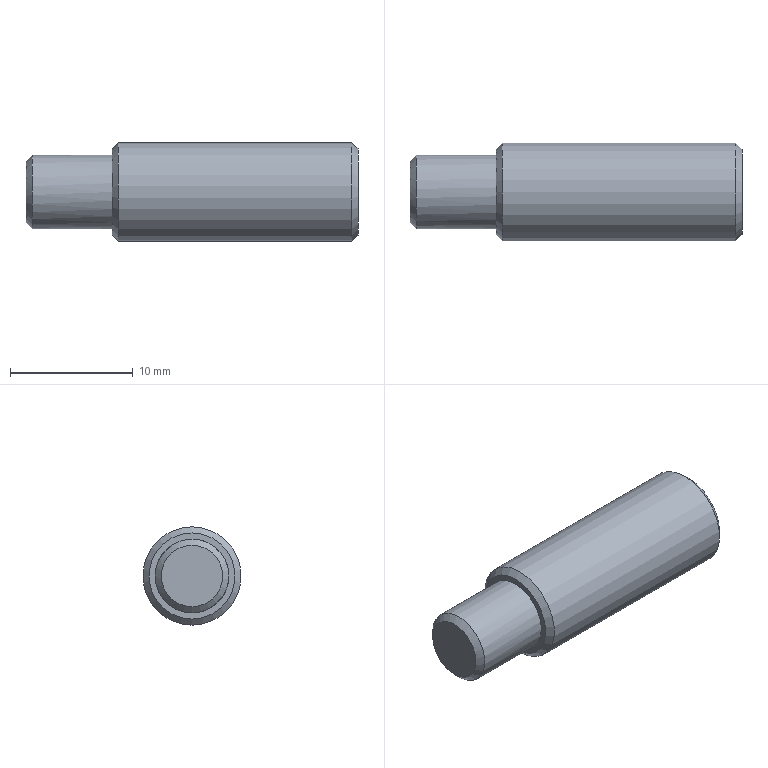Component | NX | LOC_PIN | 1 solid | 8 faces | box 27 x 8 x 8 mm | volume 1195 mm3 | plane 3 | cone 3 | cylinder 2 | commonest cylinder face diameters 6 x1 8 x1
STEP:
#1=CARTESIAN_POINT('',(0.,0.,0.));
#2=DIRECTION('',(0.,0.,1.));
#3=DIRECTION('',(1.,0.,0.));
#4=AXIS2_PLACEMENT_3D('',#1,#2,#3);
#5=CARTESIAN_POINT('',(-29.5,0.,-42.));
#6=VERTEX_POINT('',#5);
#7=CARTESIAN_POINT('',(-29.5,3.,-39.));
#8=VERTEX_POINT('',#7);
#9=CARTESIAN_POINT('',(-29.5,0.,-39.));
#10=DIRECTION('',(1.,0.,0.));
#11=DIRECTION('',(0.,0.,-1.));
#12=AXIS2_PLACEMENT_3D('',#9,#10,#11);
#13=CIRCLE('',#12,3.);
#14=CARTESIAN_POINT('',(-23.,0.,-39.));
#15=DIRECTION('',(-1.,0.,0.));
#16=DIRECTION('',(0.,0.,1.));
#17=AXIS2_PLACEMENT_3D('',#14,#15,#16);
#18=CYLINDRICAL_SURFACE('',#17,3.);
#19=CARTESIAN_POINT('',(3.142,6.5));
#20=DIRECTION('',(-1.,0.));
#21=VECTOR('',#20,1.);
#22=LINE('',#19,#21);
#23=(GEOMETRIC_REPRESENTATION_CONTEXT(2)PARAMETRIC_REPRESENTATION_CONTEXT()REPRESENTATION_CONTEXT('',''));
#24=DEFINITIONAL_REPRESENTATION('',(#22),#23);
#25=PCURVE('',#18,#24);
#26=CARTESIAN_POINT('',(-29.5,0.,-39.));
#27=DIRECTION('',(1.,0.,0.));
#28=DIRECTION('',(0.,0.,-1.));
#29=AXIS2_PLACEMENT_3D('',#26,#27,#28);
#30=CONICAL_SURFACE('',#29,3.,0.7854);
#31=CARTESIAN_POINT('',(0.,0.));
#32=DIRECTION('',(1.,0.));
#33=VECTOR('',#32,1.);
#34=LINE('',#31,#33);
#35=(GEOMETRIC_REPRESENTATION_CONTEXT(2)PARAMETRIC_REPRESENTATION_CONTEXT()REPRESENTATION_CONTEXT('',''));
#36=DEFINITIONAL_REPRESENTATION('',(#34),#35);
#37=PCURVE('',#30,#36);
#38=SURFACE_CURVE('',#13,(#25,#37),.PCURVE_S1.);
#39=EDGE_CURVE('',#6,#8,#38,.T.);
#40=ORIENTED_EDGE('',*,*,#39,.T.);
#41=CARTESIAN_POINT('',(-23.,3.,-39.));
#42=VERTEX_POINT('',#41);
#43=CARTESIAN_POINT('',(-23.,3.,-39.));
#44=CARTESIAN_POINT('',(-29.5,3.,-39.));
#45=B_SPLINE_CURVE_WITH_KNOTS('',1,(#43,#44),.UNSPECIFIED.,.F.,.F.,(2,2),(0.,6.5),.PIECEWISE_BEZIER_KNOTS.);
#46=CARTESIAN_POINT('',(1.571,0.));
#47=DIRECTION('',(0.,1.));
#48=VECTOR('',#47,1.);
#49=LINE('',#46,#48);
#50=(GEOMETRIC_REPRESENTATION_CONTEXT(2)PARAMETRIC_REPRESENTATION_CONTEXT()REPRESENTATION_CONTEXT('',''));
#51=DEFINITIONAL_REPRESENTATION('',(#49),#50);
#52=PCURVE('',#18,#51);
#53=CARTESIAN_POINT('',(7.854,0.));
#54=DIRECTION('',(0.,1.));
#55=VECTOR('',#54,1.);
#56=LINE('',#53,#55);
#57=(GEOMETRIC_REPRESENTATION_CONTEXT(2)PARAMETRIC_REPRESENTATION_CONTEXT()REPRESENTATION_CONTEXT('',''));
#58=DEFINITIONAL_REPRESENTATION('',(#56),#57);
#59=PCURVE('',#18,#58);
#60=SEAM_CURVE('',#45,(#52,#59),.PCURVE_S1.);
#61=EDGE_CURVE('',#42,#8,#60,.T.);
#62=ORIENTED_EDGE('',*,*,#61,.F.);
#63=CARTESIAN_POINT('',(-23.,0.,-39.));
#64=DIRECTION('',(1.,0.,0.));
#65=DIRECTION('',(0.,1.,0.));
#66=AXIS2_PLACEMENT_3D('',#63,#64,#65);
#67=CIRCLE('',#66,3.);
#68=CARTESIAN_POINT('',(7.854,0.));
#69=DIRECTION('',(-1.,0.));
#70=VECTOR('',#69,1.);
#71=LINE('',#68,#70);
#72=(GEOMETRIC_REPRESENTATION_CONTEXT(2)PARAMETRIC_REPRESENTATION_CONTEXT()REPRESENTATION_CONTEXT('',''));
#73=DEFINITIONAL_REPRESENTATION('',(#71),#72);
#74=PCURVE('',#18,#73);
#75=CARTESIAN_POINT('',(-23.,0.,-39.));
#76=DIRECTION('',(1.,0.,0.));
#77=DIRECTION('',(0.,0.,-1.));
#78=AXIS2_PLACEMENT_3D('',#75,#76,#77);
#79=PLANE('',#78);
#80=CARTESIAN_POINT('',(0.,0.));
#81=DIRECTION('',(0.,1.));
#82=AXIS2_PLACEMENT_2D('',#80,#81);
#83=CIRCLE('',#82,3.);
#84=(GEOMETRIC_REPRESENTATION_CONTEXT(2)PARAMETRIC_REPRESENTATION_CONTEXT()REPRESENTATION_CONTEXT('',''));
#85=DEFINITIONAL_REPRESENTATION('',(#83),#84);
#86=PCURVE('',#79,#85);
#87=SURFACE_CURVE('',#67,(#74,#86),.PCURVE_S1.);
#88=EDGE_CURVE('',#42,#42,#87,.T.);
#89=ORIENTED_EDGE('',*,*,#88,.F.);
#90=ORIENTED_EDGE('',*,*,#61,.T.);
#91=CARTESIAN_POINT('',(-29.5,0.,-39.));
#92=DIRECTION('',(1.,0.,0.));
#93=DIRECTION('',(0.,0.,-1.));
#94=AXIS2_PLACEMENT_3D('',#91,#92,#93);
#95=CIRCLE('',#94,3.);
#96=CARTESIAN_POINT('',(9.425,6.5));
#97=DIRECTION('',(-1.,0.));
#98=VECTOR('',#97,1.);
#99=LINE('',#96,#98);
#100=(GEOMETRIC_REPRESENTATION_CONTEXT(2)PARAMETRIC_REPRESENTATION_CONTEXT()REPRESENTATION_CONTEXT('',''));
#101=DEFINITIONAL_REPRESENTATION('',(#99),#100);
#102=PCURVE('',#18,#101);
#103=CARTESIAN_POINT('',(0.,0.));
#104=DIRECTION('',(1.,0.));
#105=VECTOR('',#104,1.);
#106=LINE('',#103,#105);
#107=(GEOMETRIC_REPRESENTATION_CONTEXT(2)PARAMETRIC_REPRESENTATION_CONTEXT()REPRESENTATION_CONTEXT('',''));
#108=DEFINITIONAL_REPRESENTATION('',(#106),#107);
#109=PCURVE('',#30,#108);
#110=SURFACE_CURVE('',#95,(#102,#109),.PCURVE_S1.);
#111=EDGE_CURVE('',#8,#6,#110,.T.);
#112=ORIENTED_EDGE('',*,*,#111,.T.);
#113=EDGE_LOOP('',(#40,#62,#89,#90,#112));
#114=FACE_BOUND('',#113,.T.);
#115=ADVANCED_FACE('',(#114),#18,.T.);
#116=CARTESIAN_POINT('',(-30.,0.,-41.5));
#117=VERTEX_POINT('',#116);
#118=CARTESIAN_POINT('',(-30.,0.,-39.));
#119=DIRECTION('',(-1.,0.,0.));
#120=DIRECTION('',(0.,0.,-1.));
#121=AXIS2_PLACEMENT_3D('',#118,#119,#120);
#122=CIRCLE('',#121,2.5);
#123=CARTESIAN_POINT('',(-30.,0.,-39.));
#124=DIRECTION('',(1.,0.,0.));
#125=DIRECTION('',(0.,0.,-1.));
#126=AXIS2_PLACEMENT_3D('',#123,#124,#125);
#127=PLANE('',#126);
#128=CARTESIAN_POINT('',(2.5,0.));
#129=CARTESIAN_POINT('',(2.5,-4.33));
#130=CARTESIAN_POINT('',(-1.25,-2.165));
#131=CARTESIAN_POINT('',(-5.,-0.));
#132=CARTESIAN_POINT('',(-1.25,2.165));
#133=CARTESIAN_POINT('',(2.5,4.33));
#134=CARTESIAN_POINT('',(2.5,0.));
#135=(BOUNDED_CURVE()B_SPLINE_CURVE(2,(#128,#129,#130,#131,#132,#133,#134),.UNSPECIFIED.,.T.,.F.)B_SPLINE_CURVE_WITH_KNOTS((1,2,2,2,2,1),(-2.094,0.,2.094,4.189,6.283,8.378),.UNSPECIFIED.)CURVE()GEOMETRIC_REPRESENTATION_ITEM()RATIONAL_B_SPLINE_CURVE((1.,0.5,1.,0.5,1.,0.5,1.))REPRESENTATION_ITEM(''));
#136=(GEOMETRIC_REPRESENTATION_CONTEXT(2)PARAMETRIC_REPRESENTATION_CONTEXT()REPRESENTATION_CONTEXT('',''));
#137=DEFINITIONAL_REPRESENTATION('',(#135),#136);
#138=PCURVE('',#127,#137);
#139=CARTESIAN_POINT('',(6.283,-0.5));
#140=DIRECTION('',(-1.,0.));
#141=VECTOR('',#140,1.);
#142=LINE('',#139,#141);
#143=(GEOMETRIC_REPRESENTATION_CONTEXT(2)PARAMETRIC_REPRESENTATION_CONTEXT()REPRESENTATION_CONTEXT('',''));
#144=DEFINITIONAL_REPRESENTATION('',(#142),#143);
#145=PCURVE('',#30,#144);
#146=SURFACE_CURVE('',#122,(#138,#145),.PCURVE_S1.);
#147=EDGE_CURVE('',#117,#117,#146,.T.);
#148=ORIENTED_EDGE('',*,*,#147,.T.);
#149=EDGE_LOOP('',(#148));
#150=FACE_BOUND('',#149,.T.);
#151=ADVANCED_FACE('',(#150),#127,.F.);
#152=CARTESIAN_POINT('',(-22.5,0.,-43.));
#153=VERTEX_POINT('',#152);
#154=CARTESIAN_POINT('',(-22.5,0.,-39.));
#155=DIRECTION('',(1.,0.,0.));
#156=DIRECTION('',(0.,0.,-1.));
#157=AXIS2_PLACEMENT_3D('',#154,#155,#156);
#158=CIRCLE('',#157,4.);
#159=CARTESIAN_POINT('',(-3.,0.,-39.));
#160=DIRECTION('',(-1.,0.,0.));
#161=DIRECTION('',(0.,0.,1.));
#162=AXIS2_PLACEMENT_3D('',#159,#160,#161);
#163=CYLINDRICAL_SURFACE('',#162,4.);
#164=CARTESIAN_POINT('',(9.425,19.5));
#165=DIRECTION('',(-1.,0.));
#166=VECTOR('',#165,1.);
#167=LINE('',#164,#166);
#168=(GEOMETRIC_REPRESENTATION_CONTEXT(2)PARAMETRIC_REPRESENTATION_CONTEXT()REPRESENTATION_CONTEXT('',''));
#169=DEFINITIONAL_REPRESENTATION('',(#167),#168);
#170=PCURVE('',#163,#169);
#171=CARTESIAN_POINT('',(-22.5,0.,-39.));
#172=DIRECTION('',(1.,0.,0.));
#173=DIRECTION('',(0.,0.,-1.));
#174=AXIS2_PLACEMENT_3D('',#171,#172,#173);
#175=CONICAL_SURFACE('',#174,4.,0.7854);
#176=CARTESIAN_POINT('',(0.,0.));
#177=DIRECTION('',(1.,0.));
#178=VECTOR('',#177,1.);
#179=LINE('',#176,#178);
#180=(GEOMETRIC_REPRESENTATION_CONTEXT(2)PARAMETRIC_REPRESENTATION_CONTEXT()REPRESENTATION_CONTEXT('',''));
#181=DEFINITIONAL_REPRESENTATION('',(#179),#180);
#182=PCURVE('',#175,#181);
#183=SURFACE_CURVE('',#158,(#170,#182),.PCURVE_S1.);
#184=EDGE_CURVE('',#153,#153,#183,.T.);
#185=ORIENTED_EDGE('',*,*,#184,.T.);
#186=CARTESIAN_POINT('',(-3.5,0.,-43.));
#187=VERTEX_POINT('',#186);
#188=CARTESIAN_POINT('',(-3.5,0.,-43.));
#189=CARTESIAN_POINT('',(-22.5,0.,-43.));
#190=B_SPLINE_CURVE_WITH_KNOTS('',1,(#188,#189),.UNSPECIFIED.,.F.,.F.,(2,2),(0.5,19.5),.PIECEWISE_BEZIER_KNOTS.);
#191=CARTESIAN_POINT('',(3.142,0.));
#192=DIRECTION('',(0.,1.));
#193=VECTOR('',#192,1.);
#194=LINE('',#191,#193);
#195=(GEOMETRIC_REPRESENTATION_CONTEXT(2)PARAMETRIC_REPRESENTATION_CONTEXT()REPRESENTATION_CONTEXT('',''));
#196=DEFINITIONAL_REPRESENTATION('',(#194),#195);
#197=PCURVE('',#163,#196);
#198=CARTESIAN_POINT('',(9.425,0.));
#199=DIRECTION('',(0.,1.));
#200=VECTOR('',#199,1.);
#201=LINE('',#198,#200);
#202=(GEOMETRIC_REPRESENTATION_CONTEXT(2)PARAMETRIC_REPRESENTATION_CONTEXT()REPRESENTATION_CONTEXT('',''));
#203=DEFINITIONAL_REPRESENTATION('',(#201),#202);
#204=PCURVE('',#163,#203);
#205=SEAM_CURVE('',#190,(#197,#204),.PCURVE_S1.);
#206=EDGE_CURVE('',#187,#153,#205,.T.);
#207=ORIENTED_EDGE('',*,*,#206,.F.);
#208=CARTESIAN_POINT('',(-3.5,0.,-39.));
#209=DIRECTION('',(-1.,0.,0.));
#210=DIRECTION('',(0.,0.,-1.));
#211=AXIS2_PLACEMENT_3D('',#208,#209,#210);
#212=CIRCLE('',#211,4.);
#213=CARTESIAN_POINT('',(3.142,0.5));
#214=DIRECTION('',(1.,0.));
#215=VECTOR('',#214,1.);
#216=LINE('',#213,#215);
#217=(GEOMETRIC_REPRESENTATION_CONTEXT(2)PARAMETRIC_REPRESENTATION_CONTEXT()REPRESENTATION_CONTEXT('',''));
#218=DEFINITIONAL_REPRESENTATION('',(#216),#217);
#219=PCURVE('',#163,#218);
#220=CARTESIAN_POINT('',(-3.,0.,-39.));
#221=DIRECTION('',(-1.,0.,0.));
#222=DIRECTION('',(0.,0.,1.));
#223=AXIS2_PLACEMENT_3D('',#220,#221,#222);
#224=CONICAL_SURFACE('',#223,3.5,0.7854);
#225=CARTESIAN_POINT('',(3.142,0.5));
#226=DIRECTION('',(1.,0.));
#227=VECTOR('',#226,1.);
#228=LINE('',#225,#227);
#229=(GEOMETRIC_REPRESENTATION_CONTEXT(2)PARAMETRIC_REPRESENTATION_CONTEXT()REPRESENTATION_CONTEXT('',''));
#230=DEFINITIONAL_REPRESENTATION('',(#228),#229);
#231=PCURVE('',#224,#230);
#232=SURFACE_CURVE('',#212,(#219,#231),.PCURVE_S1.);
#233=EDGE_CURVE('',#187,#187,#232,.T.);
#234=ORIENTED_EDGE('',*,*,#233,.T.);
#235=ORIENTED_EDGE('',*,*,#206,.T.);
#236=EDGE_LOOP('',(#185,#207,#234,#235));
#237=FACE_BOUND('',#236,.T.);
#238=ADVANCED_FACE('',(#237),#163,.T.);
#239=CARTESIAN_POINT('',(-3.,0.,-42.5));
#240=VERTEX_POINT('',#239);
#241=CARTESIAN_POINT('',(-3.,0.,-39.));
#242=DIRECTION('',(1.,0.,0.));
#243=DIRECTION('',(0.,0.,-1.));
#244=AXIS2_PLACEMENT_3D('',#241,#242,#243);
#245=CIRCLE('',#244,3.5);
#246=CARTESIAN_POINT('',(-3.,0.,-39.));
#247=DIRECTION('',(1.,0.,0.));
#248=DIRECTION('',(0.,0.,-1.));
#249=AXIS2_PLACEMENT_3D('',#246,#247,#248);
#250=PLANE('',#249);
#251=CARTESIAN_POINT('',(0.,0.));
#252=DIRECTION('',(1.,0.));
#253=AXIS2_PLACEMENT_2D('',#251,#252);
#254=CIRCLE('',#253,3.5);
#255=(GEOMETRIC_REPRESENTATION_CONTEXT(2)PARAMETRIC_REPRESENTATION_CONTEXT()REPRESENTATION_CONTEXT('',''));
#256=DEFINITIONAL_REPRESENTATION('',(#254),#255);
#257=PCURVE('',#250,#256);
#258=CARTESIAN_POINT('',(9.425,0.));
#259=DIRECTION('',(-1.,0.));
#260=VECTOR('',#259,1.);
#261=LINE('',#258,#260);
#262=(GEOMETRIC_REPRESENTATION_CONTEXT(2)PARAMETRIC_REPRESENTATION_CONTEXT()REPRESENTATION_CONTEXT('',''));
#263=DEFINITIONAL_REPRESENTATION('',(#261),#262);
#264=PCURVE('',#224,#263);
#265=SURFACE_CURVE('',#245,(#257,#264),.PCURVE_S1.);
#266=EDGE_CURVE('',#240,#240,#265,.T.);
#267=ORIENTED_EDGE('',*,*,#266,.T.);
#268=EDGE_LOOP('',(#267));
#269=FACE_BOUND('',#268,.T.);
#270=ADVANCED_FACE('',(#269),#250,.T.);
#271=CARTESIAN_POINT('',(-23.,0.,-42.5));
#272=VERTEX_POINT('',#271);
#273=CARTESIAN_POINT('',(-23.,0.,-39.));
#274=DIRECTION('',(-1.,0.,0.));
#275=DIRECTION('',(0.,0.,-1.));
#276=AXIS2_PLACEMENT_3D('',#273,#274,#275);
#277=CIRCLE('',#276,3.5);
#278=CARTESIAN_POINT('',(3.5,0.));
#279=CARTESIAN_POINT('',(3.5,-6.062));
#280=CARTESIAN_POINT('',(-1.75,-3.031));
#281=CARTESIAN_POINT('',(-7.,-0.));
#282=CARTESIAN_POINT('',(-1.75,3.031));
#283=CARTESIAN_POINT('',(3.5,6.062));
#284=CARTESIAN_POINT('',(3.5,0.));
#285=(BOUNDED_CURVE()B_SPLINE_CURVE(2,(#278,#279,#280,#281,#282,#283,#284),.UNSPECIFIED.,.T.,.F.)B_SPLINE_CURVE_WITH_KNOTS((1,2,2,2,2,1),(-2.094,0.,2.094,4.189,6.283,8.378),.UNSPECIFIED.)CURVE()GEOMETRIC_REPRESENTATION_ITEM()RATIONAL_B_SPLINE_CURVE((1.,0.5,1.,0.5,1.,0.5,1.))REPRESENTATION_ITEM(''));
#286=(GEOMETRIC_REPRESENTATION_CONTEXT(2)PARAMETRIC_REPRESENTATION_CONTEXT()REPRESENTATION_CONTEXT('',''));
#287=DEFINITIONAL_REPRESENTATION('',(#285),#286);
#288=PCURVE('',#79,#287);
#289=CARTESIAN_POINT('',(6.283,-0.5));
#290=DIRECTION('',(-1.,0.));
#291=VECTOR('',#290,1.);
#292=LINE('',#289,#291);
#293=(GEOMETRIC_REPRESENTATION_CONTEXT(2)PARAMETRIC_REPRESENTATION_CONTEXT()REPRESENTATION_CONTEXT('',''));
#294=DEFINITIONAL_REPRESENTATION('',(#292),#293);
#295=PCURVE('',#175,#294);
#296=SURFACE_CURVE('',#277,(#288,#295),.PCURVE_S1.);
#297=EDGE_CURVE('',#272,#272,#296,.T.);
#298=ORIENTED_EDGE('',*,*,#297,.T.);
#299=EDGE_LOOP('',(#298));
#300=FACE_BOUND('',#299,.T.);
#301=ORIENTED_EDGE('',*,*,#88,.T.);
#302=EDGE_LOOP('',(#301));
#303=FACE_BOUND('',#302,.T.);
#304=ADVANCED_FACE('',(#300,#303),#79,.F.);
#305=ORIENTED_EDGE('',*,*,#147,.F.);
#306=CARTESIAN_POINT('',(-30.,0.,-41.5));
#307=CARTESIAN_POINT('',(-29.5,0.,-42.));
#308=B_SPLINE_CURVE_WITH_KNOTS('',1,(#306,#307),.UNSPECIFIED.,.F.,.F.,(2,2),(-0.7071,0.),.PIECEWISE_BEZIER_KNOTS.);
#309=CARTESIAN_POINT('',(6.283,0.));
#310=DIRECTION('',(0.,1.));
#311=VECTOR('',#310,1.);
#312=LINE('',#309,#311);
#313=(GEOMETRIC_REPRESENTATION_CONTEXT(2)PARAMETRIC_REPRESENTATION_CONTEXT()REPRESENTATION_CONTEXT('',''));
#314=DEFINITIONAL_REPRESENTATION('',(#312),#313);
#315=PCURVE('',#30,#314);
#316=CARTESIAN_POINT('',(0.,0.));
#317=DIRECTION('',(0.,1.));
#318=VECTOR('',#317,1.);
#319=LINE('',#316,#318);
#320=(GEOMETRIC_REPRESENTATION_CONTEXT(2)PARAMETRIC_REPRESENTATION_CONTEXT()REPRESENTATION_CONTEXT('',''));
#321=DEFINITIONAL_REPRESENTATION('',(#319),#320);
#322=PCURVE('',#30,#321);
#323=SEAM_CURVE('',#308,(#315,#322),.PCURVE_S1.);
#324=EDGE_CURVE('',#117,#6,#323,.T.);
#325=ORIENTED_EDGE('',*,*,#324,.T.);
#326=ORIENTED_EDGE('',*,*,#111,.F.);
#327=ORIENTED_EDGE('',*,*,#39,.F.);
#328=ORIENTED_EDGE('',*,*,#324,.F.);
#329=EDGE_LOOP('',(#305,#325,#326,#327,#328));
#330=FACE_BOUND('',#329,.T.);
#331=ADVANCED_FACE('',(#330),#30,.T.);
#332=ORIENTED_EDGE('',*,*,#297,.F.);
#333=CARTESIAN_POINT('',(-23.,0.,-42.5));
#334=CARTESIAN_POINT('',(-22.5,0.,-43.));
#335=B_SPLINE_CURVE_WITH_KNOTS('',1,(#333,#334),.UNSPECIFIED.,.F.,.F.,(2,2),(-0.7071,0.),.PIECEWISE_BEZIER_KNOTS.);
#336=CARTESIAN_POINT('',(6.283,0.));
#337=DIRECTION('',(0.,1.));
#338=VECTOR('',#337,1.);
#339=LINE('',#336,#338);
#340=(GEOMETRIC_REPRESENTATION_CONTEXT(2)PARAMETRIC_REPRESENTATION_CONTEXT()REPRESENTATION_CONTEXT('',''));
#341=DEFINITIONAL_REPRESENTATION('',(#339),#340);
#342=PCURVE('',#175,#341);
#343=CARTESIAN_POINT('',(0.,0.));
#344=DIRECTION('',(0.,1.));
#345=VECTOR('',#344,1.);
#346=LINE('',#343,#345);
#347=(GEOMETRIC_REPRESENTATION_CONTEXT(2)PARAMETRIC_REPRESENTATION_CONTEXT()REPRESENTATION_CONTEXT('',''));
#348=DEFINITIONAL_REPRESENTATION('',(#346),#347);
#349=PCURVE('',#175,#348);
#350=SEAM_CURVE('',#335,(#342,#349),.PCURVE_S1.);
#351=EDGE_CURVE('',#272,#153,#350,.T.);
#352=ORIENTED_EDGE('',*,*,#351,.T.);
#353=ORIENTED_EDGE('',*,*,#184,.F.);
#354=ORIENTED_EDGE('',*,*,#351,.F.);
#355=EDGE_LOOP('',(#332,#352,#353,#354));
#356=FACE_BOUND('',#355,.T.);
#357=ADVANCED_FACE('',(#356),#175,.T.);
#358=ORIENTED_EDGE('',*,*,#233,.F.);
#359=CARTESIAN_POINT('',(-3.,0.,-42.5));
#360=CARTESIAN_POINT('',(-3.5,0.,-43.));
#361=B_SPLINE_CURVE_WITH_KNOTS('',1,(#359,#360),.UNSPECIFIED.,.F.,.F.,(2,2),(0.,0.7071),.PIECEWISE_BEZIER_KNOTS.);
#362=CARTESIAN_POINT('',(3.142,0.));
#363=DIRECTION('',(0.,1.));
#364=VECTOR('',#363,1.);
#365=LINE('',#362,#364);
#366=(GEOMETRIC_REPRESENTATION_CONTEXT(2)PARAMETRIC_REPRESENTATION_CONTEXT()REPRESENTATION_CONTEXT('',''));
#367=DEFINITIONAL_REPRESENTATION('',(#365),#366);
#368=PCURVE('',#224,#367);
#369=CARTESIAN_POINT('',(9.425,0.));
#370=DIRECTION('',(0.,1.));
#371=VECTOR('',#370,1.);
#372=LINE('',#369,#371);
#373=(GEOMETRIC_REPRESENTATION_CONTEXT(2)PARAMETRIC_REPRESENTATION_CONTEXT()REPRESENTATION_CONTEXT('',''));
#374=DEFINITIONAL_REPRESENTATION('',(#372),#373);
#375=PCURVE('',#224,#374);
#376=SEAM_CURVE('',#361,(#368,#375),.PCURVE_S1.);
#377=EDGE_CURVE('',#240,#187,#376,.T.);
#378=ORIENTED_EDGE('',*,*,#377,.F.);
#379=ORIENTED_EDGE('',*,*,#266,.F.);
#380=ORIENTED_EDGE('',*,*,#377,.T.);
#381=EDGE_LOOP('',(#358,#378,#379,#380));
#382=FACE_BOUND('',#381,.T.);
#383=ADVANCED_FACE('',(#382),#224,.T.);
#384=CLOSED_SHELL('',(#115,#151,#238,#270,#304,#331,#357,#383));
#385=MANIFOLD_SOLID_BREP('',#384);
#386=(LENGTH_UNIT()NAMED_UNIT(*)SI_UNIT(.MILLI.,.METRE.));
#387=UNCERTAINTY_MEASURE_WITH_UNIT(LENGTH_MEASURE(0.00001),#386,'','');
#388=(NAMED_UNIT(*)PLANE_ANGLE_UNIT()SI_UNIT($,.RADIAN.));
#389=(NAMED_UNIT(*)SI_UNIT($,.STERADIAN.)SOLID_ANGLE_UNIT());
#390=(GEOMETRIC_REPRESENTATION_CONTEXT(3)GLOBAL_UNCERTAINTY_ASSIGNED_CONTEXT((#387))GLOBAL_UNIT_ASSIGNED_CONTEXT((#386,#388,#389))REPRESENTATION_CONTEXT('',''));
#391=ADVANCED_BREP_SHAPE_REPRESENTATION('',(#4,#385),#390);